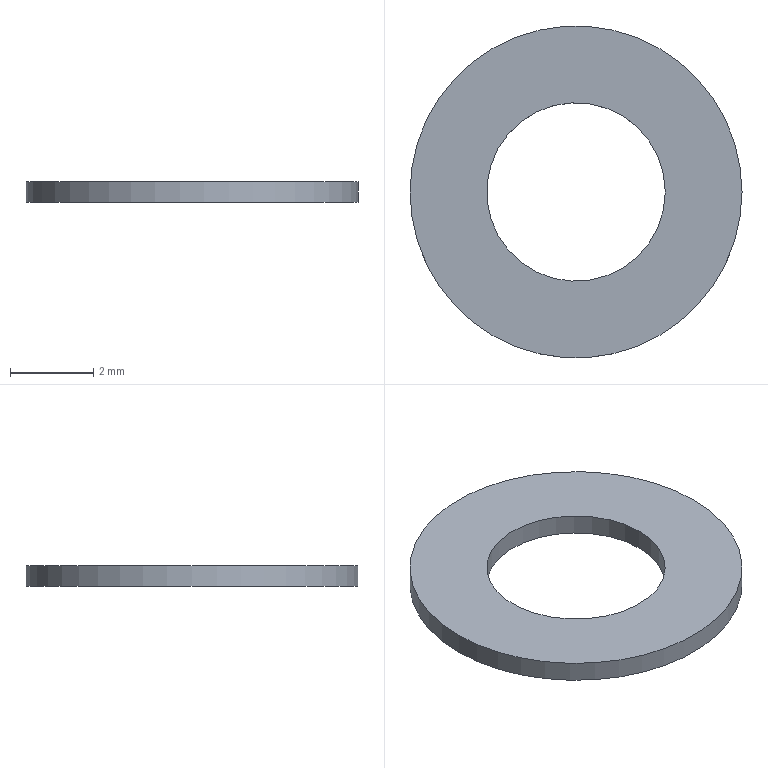Component | NX | WASHER_M4 | 1 solid | 4 faces | box 8 x 8 x 0.5 mm | volume 18 mm3 | cylinder 2 | plane 2 | commonest cylinder face diameters 8 x1 4.3 x1
STEP:
#1=CARTESIAN_POINT('',(0.,0.,0.));
#2=DIRECTION('',(0.,0.,1.));
#3=DIRECTION('',(1.,0.,0.));
#4=AXIS2_PLACEMENT_3D('',#1,#2,#3);
#5=CARTESIAN_POINT('',(-142.777,0.,294.586));
#6=VERTEX_POINT('',#5);
#7=CARTESIAN_POINT('',(-146.777,0.,294.586));
#8=DIRECTION('',(0.,0.,1.));
#9=DIRECTION('',(1.,0.,0.));
#10=AXIS2_PLACEMENT_3D('',#7,#8,#9);
#11=CIRCLE('',#10,4.);
#12=CARTESIAN_POINT('',(-146.777,0.,294.586));
#13=DIRECTION('',(0.,0.,-1.));
#14=DIRECTION('',(-1.,0.,0.));
#15=AXIS2_PLACEMENT_3D('',#12,#13,#14);
#16=CYLINDRICAL_SURFACE('',#15,4.);
#17=CARTESIAN_POINT('',(9.425,0.));
#18=DIRECTION('',(-1.,0.));
#19=VECTOR('',#18,1.);
#20=LINE('',#17,#19);
#21=(GEOMETRIC_REPRESENTATION_CONTEXT(2)PARAMETRIC_REPRESENTATION_CONTEXT()REPRESENTATION_CONTEXT('',''));
#22=DEFINITIONAL_REPRESENTATION('',(#20),#21);
#23=PCURVE('',#16,#22);
#24=CARTESIAN_POINT('',(-146.777,0.,294.586));
#25=DIRECTION('',(0.,0.,1.));
#26=DIRECTION('',(1.,0.,0.));
#27=AXIS2_PLACEMENT_3D('',#24,#25,#26);
#28=PLANE('',#27);
#29=CARTESIAN_POINT('',(0.,0.));
#30=DIRECTION('',(1.,0.));
#31=AXIS2_PLACEMENT_2D('',#29,#30);
#32=CIRCLE('',#31,4.);
#33=(GEOMETRIC_REPRESENTATION_CONTEXT(2)PARAMETRIC_REPRESENTATION_CONTEXT()REPRESENTATION_CONTEXT('',''));
#34=DEFINITIONAL_REPRESENTATION('',(#32),#33);
#35=PCURVE('',#28,#34);
#36=SURFACE_CURVE('',#11,(#23,#35),.PCURVE_S1.);
#37=EDGE_CURVE('',#6,#6,#36,.T.);
#38=ORIENTED_EDGE('',*,*,#37,.F.);
#39=CARTESIAN_POINT('',(-142.777,0.,294.086));
#40=VERTEX_POINT('',#39);
#41=CARTESIAN_POINT('',(-142.777,0.,294.586));
#42=CARTESIAN_POINT('',(-142.777,0.,294.086));
#43=B_SPLINE_CURVE_WITH_KNOTS('',1,(#41,#42),.UNSPECIFIED.,.F.,.F.,(2,2),(0.,0.5),.PIECEWISE_BEZIER_KNOTS.);
#44=CARTESIAN_POINT('',(9.425,0.));
#45=DIRECTION('',(0.,1.));
#46=VECTOR('',#45,1.);
#47=LINE('',#44,#46);
#48=(GEOMETRIC_REPRESENTATION_CONTEXT(2)PARAMETRIC_REPRESENTATION_CONTEXT()REPRESENTATION_CONTEXT('',''));
#49=DEFINITIONAL_REPRESENTATION('',(#47),#48);
#50=PCURVE('',#16,#49);
#51=CARTESIAN_POINT('',(3.142,0.));
#52=DIRECTION('',(0.,1.));
#53=VECTOR('',#52,1.);
#54=LINE('',#51,#53);
#55=(GEOMETRIC_REPRESENTATION_CONTEXT(2)PARAMETRIC_REPRESENTATION_CONTEXT()REPRESENTATION_CONTEXT('',''));
#56=DEFINITIONAL_REPRESENTATION('',(#54),#55);
#57=PCURVE('',#16,#56);
#58=SEAM_CURVE('',#43,(#50,#57),.PCURVE_S1.);
#59=EDGE_CURVE('',#6,#40,#58,.T.);
#60=ORIENTED_EDGE('',*,*,#59,.T.);
#61=CARTESIAN_POINT('',(-146.777,0.,294.086));
#62=DIRECTION('',(0.,0.,1.));
#63=DIRECTION('',(1.,0.,0.));
#64=AXIS2_PLACEMENT_3D('',#61,#62,#63);
#65=CIRCLE('',#64,4.);
#66=CARTESIAN_POINT('',(9.425,0.5));
#67=DIRECTION('',(-1.,0.));
#68=VECTOR('',#67,1.);
#69=LINE('',#66,#68);
#70=(GEOMETRIC_REPRESENTATION_CONTEXT(2)PARAMETRIC_REPRESENTATION_CONTEXT()REPRESENTATION_CONTEXT('',''));
#71=DEFINITIONAL_REPRESENTATION('',(#69),#70);
#72=PCURVE('',#16,#71);
#73=CARTESIAN_POINT('',(-146.777,0.,294.086));
#74=DIRECTION('',(0.,0.,1.));
#75=DIRECTION('',(1.,0.,0.));
#76=AXIS2_PLACEMENT_3D('',#73,#74,#75);
#77=PLANE('',#76);
#78=CARTESIAN_POINT('',(0.,0.));
#79=DIRECTION('',(1.,0.));
#80=AXIS2_PLACEMENT_2D('',#78,#79);
#81=CIRCLE('',#80,4.);
#82=(GEOMETRIC_REPRESENTATION_CONTEXT(2)PARAMETRIC_REPRESENTATION_CONTEXT()REPRESENTATION_CONTEXT('',''));
#83=DEFINITIONAL_REPRESENTATION('',(#81),#82);
#84=PCURVE('',#77,#83);
#85=SURFACE_CURVE('',#65,(#72,#84),.PCURVE_S1.);
#86=EDGE_CURVE('',#40,#40,#85,.T.);
#87=ORIENTED_EDGE('',*,*,#86,.T.);
#88=ORIENTED_EDGE('',*,*,#59,.F.);
#89=EDGE_LOOP('',(#38,#60,#87,#88));
#90=FACE_BOUND('',#89,.T.);
#91=ADVANCED_FACE('',(#90),#16,.T.);
#92=CARTESIAN_POINT('',(-144.627,0.,294.586));
#93=VERTEX_POINT('',#92);
#94=CARTESIAN_POINT('',(-146.777,0.,294.586));
#95=DIRECTION('',(0.,0.,1.));
#96=DIRECTION('',(1.,0.,0.));
#97=AXIS2_PLACEMENT_3D('',#94,#95,#96);
#98=CIRCLE('',#97,2.15);
#99=CARTESIAN_POINT('',(-146.777,0.,294.586));
#100=DIRECTION('',(0.,0.,-1.));
#101=DIRECTION('',(-1.,0.,0.));
#102=AXIS2_PLACEMENT_3D('',#99,#100,#101);
#103=CYLINDRICAL_SURFACE('',#102,2.15);
#104=CARTESIAN_POINT('',(9.425,0.));
#105=DIRECTION('',(-1.,0.));
#106=VECTOR('',#105,1.);
#107=LINE('',#104,#106);
#108=(GEOMETRIC_REPRESENTATION_CONTEXT(2)PARAMETRIC_REPRESENTATION_CONTEXT()REPRESENTATION_CONTEXT('',''));
#109=DEFINITIONAL_REPRESENTATION('',(#107),#108);
#110=PCURVE('',#103,#109);
#111=CARTESIAN_POINT('',(0.,0.));
#112=DIRECTION('',(1.,0.));
#113=AXIS2_PLACEMENT_2D('',#111,#112);
#114=CIRCLE('',#113,2.15);
#115=(GEOMETRIC_REPRESENTATION_CONTEXT(2)PARAMETRIC_REPRESENTATION_CONTEXT()REPRESENTATION_CONTEXT('',''));
#116=DEFINITIONAL_REPRESENTATION('',(#114),#115);
#117=PCURVE('',#28,#116);
#118=SURFACE_CURVE('',#98,(#110,#117),.PCURVE_S1.);
#119=EDGE_CURVE('',#93,#93,#118,.T.);
#120=ORIENTED_EDGE('',*,*,#119,.F.);
#121=CARTESIAN_POINT('',(-144.627,0.,294.086));
#122=VERTEX_POINT('',#121);
#123=CARTESIAN_POINT('',(-144.627,0.,294.586));
#124=CARTESIAN_POINT('',(-144.627,0.,294.086));
#125=B_SPLINE_CURVE_WITH_KNOTS('',1,(#123,#124),.UNSPECIFIED.,.F.,.F.,(2,2),(0.,0.5),.PIECEWISE_BEZIER_KNOTS.);
#126=CARTESIAN_POINT('',(9.425,0.));
#127=DIRECTION('',(0.,1.));
#128=VECTOR('',#127,1.);
#129=LINE('',#126,#128);
#130=(GEOMETRIC_REPRESENTATION_CONTEXT(2)PARAMETRIC_REPRESENTATION_CONTEXT()REPRESENTATION_CONTEXT('',''));
#131=DEFINITIONAL_REPRESENTATION('',(#129),#130);
#132=PCURVE('',#103,#131);
#133=CARTESIAN_POINT('',(3.142,0.));
#134=DIRECTION('',(0.,1.));
#135=VECTOR('',#134,1.);
#136=LINE('',#133,#135);
#137=(GEOMETRIC_REPRESENTATION_CONTEXT(2)PARAMETRIC_REPRESENTATION_CONTEXT()REPRESENTATION_CONTEXT('',''));
#138=DEFINITIONAL_REPRESENTATION('',(#136),#137);
#139=PCURVE('',#103,#138);
#140=SEAM_CURVE('',#125,(#132,#139),.PCURVE_S1.);
#141=EDGE_CURVE('',#93,#122,#140,.T.);
#142=ORIENTED_EDGE('',*,*,#141,.T.);
#143=CARTESIAN_POINT('',(-146.777,0.,294.086));
#144=DIRECTION('',(0.,0.,1.));
#145=DIRECTION('',(1.,0.,0.));
#146=AXIS2_PLACEMENT_3D('',#143,#144,#145);
#147=CIRCLE('',#146,2.15);
#148=CARTESIAN_POINT('',(9.425,0.5));
#149=DIRECTION('',(-1.,0.));
#150=VECTOR('',#149,1.);
#151=LINE('',#148,#150);
#152=(GEOMETRIC_REPRESENTATION_CONTEXT(2)PARAMETRIC_REPRESENTATION_CONTEXT()REPRESENTATION_CONTEXT('',''));
#153=DEFINITIONAL_REPRESENTATION('',(#151),#152);
#154=PCURVE('',#103,#153);
#155=CARTESIAN_POINT('',(0.,0.));
#156=DIRECTION('',(1.,0.));
#157=AXIS2_PLACEMENT_2D('',#155,#156);
#158=CIRCLE('',#157,2.15);
#159=(GEOMETRIC_REPRESENTATION_CONTEXT(2)PARAMETRIC_REPRESENTATION_CONTEXT()REPRESENTATION_CONTEXT('',''));
#160=DEFINITIONAL_REPRESENTATION('',(#158),#159);
#161=PCURVE('',#77,#160);
#162=SURFACE_CURVE('',#147,(#154,#161),.PCURVE_S1.);
#163=EDGE_CURVE('',#122,#122,#162,.T.);
#164=ORIENTED_EDGE('',*,*,#163,.T.);
#165=ORIENTED_EDGE('',*,*,#141,.F.);
#166=EDGE_LOOP('',(#120,#142,#164,#165));
#167=FACE_BOUND('',#166,.F.);
#168=ADVANCED_FACE('',(#167),#103,.F.);
#169=ORIENTED_EDGE('',*,*,#37,.T.);
#170=EDGE_LOOP('',(#169));
#171=FACE_BOUND('',#170,.T.);
#172=ORIENTED_EDGE('',*,*,#119,.F.);
#173=EDGE_LOOP('',(#172));
#174=FACE_BOUND('',#173,.T.);
#175=ADVANCED_FACE('',(#171,#174),#28,.T.);
#176=ORIENTED_EDGE('',*,*,#86,.F.);
#177=EDGE_LOOP('',(#176));
#178=FACE_BOUND('',#177,.T.);
#179=ORIENTED_EDGE('',*,*,#163,.T.);
#180=EDGE_LOOP('',(#179));
#181=FACE_BOUND('',#180,.T.);
#182=ADVANCED_FACE('',(#178,#181),#77,.F.);
#183=CLOSED_SHELL('',(#91,#168,#175,#182));
#184=MANIFOLD_SOLID_BREP('',#183);
#185=(LENGTH_UNIT()NAMED_UNIT(*)SI_UNIT(.MILLI.,.METRE.));
#186=UNCERTAINTY_MEASURE_WITH_UNIT(LENGTH_MEASURE(0.00001),#185,'','');
#187=(NAMED_UNIT(*)PLANE_ANGLE_UNIT()SI_UNIT($,.RADIAN.));
#188=(NAMED_UNIT(*)SI_UNIT($,.STERADIAN.)SOLID_ANGLE_UNIT());
#189=(GEOMETRIC_REPRESENTATION_CONTEXT(3)GLOBAL_UNCERTAINTY_ASSIGNED_CONTEXT((#186))GLOBAL_UNIT_ASSIGNED_CONTEXT((#185,#187,#188))REPRESENTATION_CONTEXT('',''));
#190=ADVANCED_BREP_SHAPE_REPRESENTATION('',(#4,#184),#189);